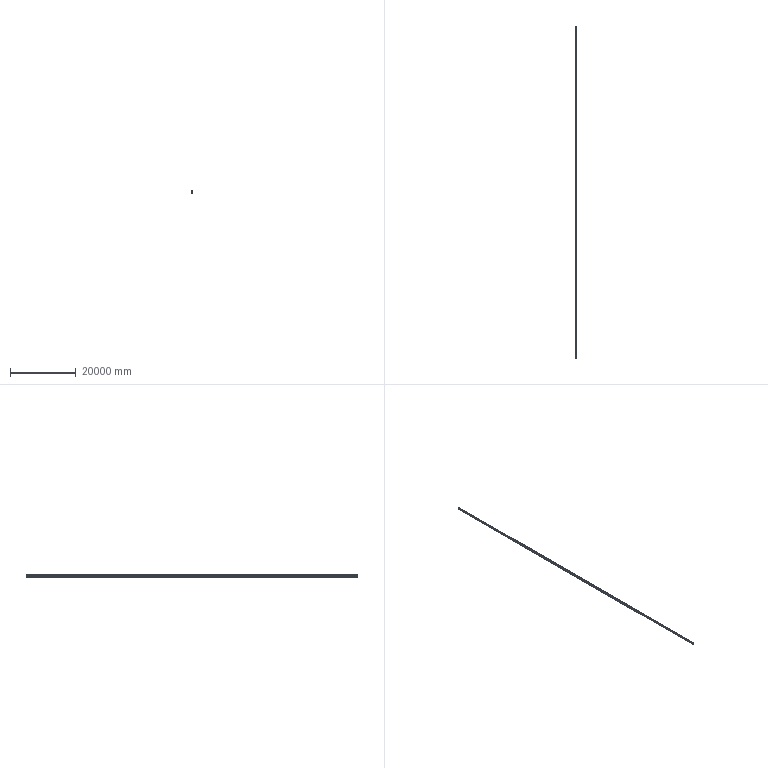Component | NX | GD | 1 solid | 14 faces | volume 1553098200 mm3 | plane 14